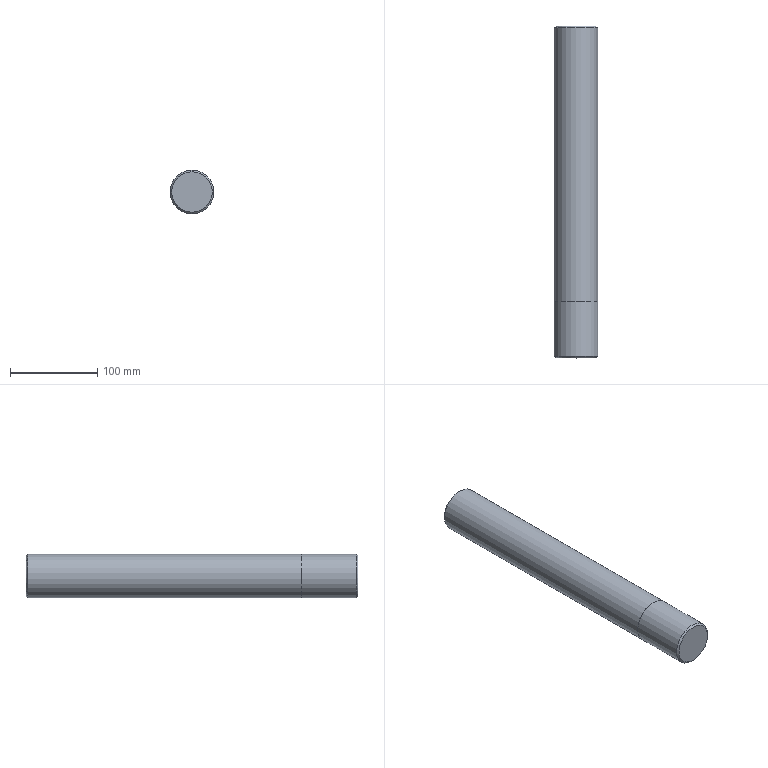Component | NX | GUIDE_PILLER | 1 solid | 7 faces | box 50.2 x 380 x 50.2 mm | volume 746538 mm3 | plane 3 | cylinder 2 | cone 2 | commonest cylinder face diameters 50.2 x1 50 x1
STEP:
#1=CARTESIAN_POINT('',(0.,0.,0.));
#2=DIRECTION('',(0.,0.,1.));
#3=DIRECTION('',(1.,0.,0.));
#4=AXIS2_PLACEMENT_3D('',#1,#2,#3);
#5=CARTESIAN_POINT('',(-120.,-68.,-232.946));
#6=VERTEX_POINT('',#5);
#7=CARTESIAN_POINT('',(-120.,-68.,-182.746));
#8=VERTEX_POINT('',#7);
#9=CARTESIAN_POINT('',(-120.,-68.,-207.846));
#10=DIRECTION('',(0.,1.,0.));
#11=DIRECTION('',(0.,0.,-1.));
#12=AXIS2_PLACEMENT_3D('',#9,#10,#11);
#13=CIRCLE('',#12,25.1);
#14=CARTESIAN_POINT('',(-120.,310.,-207.846));
#15=DIRECTION('',(0.,-1.,-0.));
#16=DIRECTION('',(0.,-0.,1.));
#17=AXIS2_PLACEMENT_3D('',#14,#15,#16);
#18=CYLINDRICAL_SURFACE('',#17,25.1);
#19=CARTESIAN_POINT('',(3.142,378.));
#20=DIRECTION('',(-1.,0.));
#21=VECTOR('',#20,1.);
#22=LINE('',#19,#21);
#23=(GEOMETRIC_REPRESENTATION_CONTEXT(2)PARAMETRIC_REPRESENTATION_CONTEXT()REPRESENTATION_CONTEXT('',''));
#24=DEFINITIONAL_REPRESENTATION('',(#22),#23);
#25=PCURVE('',#18,#24);
#26=CARTESIAN_POINT('',(-120.,-70.,-207.846));
#27=DIRECTION('',(0.,1.,0.));
#28=DIRECTION('',(0.,0.,-1.));
#29=AXIS2_PLACEMENT_3D('',#26,#27,#28);
#30=CONICAL_SURFACE('',#29,23.1,0.7854);
#31=CARTESIAN_POINT('',(0.,2.));
#32=DIRECTION('',(1.,0.));
#33=VECTOR('',#32,1.);
#34=LINE('',#31,#33);
#35=(GEOMETRIC_REPRESENTATION_CONTEXT(2)PARAMETRIC_REPRESENTATION_CONTEXT()REPRESENTATION_CONTEXT('',''));
#36=DEFINITIONAL_REPRESENTATION('',(#34),#35);
#37=PCURVE('',#30,#36);
#38=SURFACE_CURVE('',#13,(#25,#37),.PCURVE_S1.);
#39=EDGE_CURVE('',#6,#8,#38,.T.);
#40=ORIENTED_EDGE('',*,*,#39,.T.);
#41=CARTESIAN_POINT('',(-120.,-5.,-182.746));
#42=VERTEX_POINT('',#41);
#43=CARTESIAN_POINT('',(-120.,-5.,-182.746));
#44=CARTESIAN_POINT('',(-120.,-68.,-182.746));
#45=B_SPLINE_CURVE_WITH_KNOTS('',1,(#43,#44),.UNSPECIFIED.,.F.,.F.,(2,2),(315.,378.),.PIECEWISE_BEZIER_KNOTS.);
#46=CARTESIAN_POINT('',(0.,0.));
#47=DIRECTION('',(0.,1.));
#48=VECTOR('',#47,1.);
#49=LINE('',#46,#48);
#50=(GEOMETRIC_REPRESENTATION_CONTEXT(2)PARAMETRIC_REPRESENTATION_CONTEXT()REPRESENTATION_CONTEXT('',''));
#51=DEFINITIONAL_REPRESENTATION('',(#49),#50);
#52=PCURVE('',#18,#51);
#53=CARTESIAN_POINT('',(6.283,0.));
#54=DIRECTION('',(0.,1.));
#55=VECTOR('',#54,1.);
#56=LINE('',#53,#55);
#57=(GEOMETRIC_REPRESENTATION_CONTEXT(2)PARAMETRIC_REPRESENTATION_CONTEXT()REPRESENTATION_CONTEXT('',''));
#58=DEFINITIONAL_REPRESENTATION('',(#56),#57);
#59=PCURVE('',#18,#58);
#60=SEAM_CURVE('',#45,(#52,#59),.PCURVE_S1.);
#61=EDGE_CURVE('',#42,#8,#60,.T.);
#62=ORIENTED_EDGE('',*,*,#61,.F.);
#63=CARTESIAN_POINT('',(-120.,-5.,-207.846));
#64=DIRECTION('',(0.,-1.,-0.));
#65=DIRECTION('',(0.,-0.,1.));
#66=AXIS2_PLACEMENT_3D('',#63,#64,#65);
#67=CIRCLE('',#66,25.1);
#68=CARTESIAN_POINT('',(0.,315.));
#69=DIRECTION('',(1.,0.));
#70=VECTOR('',#69,1.);
#71=LINE('',#68,#70);
#72=(GEOMETRIC_REPRESENTATION_CONTEXT(2)PARAMETRIC_REPRESENTATION_CONTEXT()REPRESENTATION_CONTEXT('',''));
#73=DEFINITIONAL_REPRESENTATION('',(#71),#72);
#74=PCURVE('',#18,#73);
#75=CARTESIAN_POINT('',(-120.,-5.,-182.846));
#76=DIRECTION('',(0.,-1.,-0.));
#77=DIRECTION('',(0.,-0.,1.));
#78=AXIS2_PLACEMENT_3D('',#75,#76,#77);
#79=PLANE('',#78);
#80=CARTESIAN_POINT('',(-25.,0.));
#81=DIRECTION('',(1.,0.));
#82=AXIS2_PLACEMENT_2D('',#80,#81);
#83=CIRCLE('',#82,25.1);
#84=(GEOMETRIC_REPRESENTATION_CONTEXT(2)PARAMETRIC_REPRESENTATION_CONTEXT()REPRESENTATION_CONTEXT('',''));
#85=DEFINITIONAL_REPRESENTATION('',(#83),#84);
#86=PCURVE('',#79,#85);
#87=SURFACE_CURVE('',#67,(#74,#86),.PCURVE_S1.);
#88=EDGE_CURVE('',#42,#42,#87,.T.);
#89=ORIENTED_EDGE('',*,*,#88,.T.);
#90=ORIENTED_EDGE('',*,*,#61,.T.);
#91=CARTESIAN_POINT('',(-120.,-68.,-207.846));
#92=DIRECTION('',(0.,1.,0.));
#93=DIRECTION('',(0.,0.,-1.));
#94=AXIS2_PLACEMENT_3D('',#91,#92,#93);
#95=CIRCLE('',#94,25.1);
#96=CARTESIAN_POINT('',(9.425,378.));
#97=DIRECTION('',(-1.,0.));
#98=VECTOR('',#97,1.);
#99=LINE('',#96,#98);
#100=(GEOMETRIC_REPRESENTATION_CONTEXT(2)PARAMETRIC_REPRESENTATION_CONTEXT()REPRESENTATION_CONTEXT('',''));
#101=DEFINITIONAL_REPRESENTATION('',(#99),#100);
#102=PCURVE('',#18,#101);
#103=CARTESIAN_POINT('',(0.,2.));
#104=DIRECTION('',(1.,0.));
#105=VECTOR('',#104,1.);
#106=LINE('',#103,#105);
#107=(GEOMETRIC_REPRESENTATION_CONTEXT(2)PARAMETRIC_REPRESENTATION_CONTEXT()REPRESENTATION_CONTEXT('',''));
#108=DEFINITIONAL_REPRESENTATION('',(#106),#107);
#109=PCURVE('',#30,#108);
#110=SURFACE_CURVE('',#95,(#102,#109),.PCURVE_S1.);
#111=EDGE_CURVE('',#8,#6,#110,.T.);
#112=ORIENTED_EDGE('',*,*,#111,.T.);
#113=EDGE_LOOP('',(#40,#62,#89,#90,#112));
#114=FACE_BOUND('',#113,.T.);
#115=ADVANCED_FACE('',(#114),#18,.T.);
#116=CARTESIAN_POINT('',(-120.,-70.,-230.946));
#117=VERTEX_POINT('',#116);
#118=CARTESIAN_POINT('',(-120.,-70.,-207.846));
#119=DIRECTION('',(0.,-1.,-0.));
#120=DIRECTION('',(0.,0.,-1.));
#121=AXIS2_PLACEMENT_3D('',#118,#119,#120);
#122=CIRCLE('',#121,23.1);
#123=CARTESIAN_POINT('',(-120.,-70.,-182.746));
#124=DIRECTION('',(0.,1.,0.));
#125=DIRECTION('',(0.,0.,-1.));
#126=AXIS2_PLACEMENT_3D('',#123,#124,#125);
#127=PLANE('',#126);
#128=CARTESIAN_POINT('',(48.2,0.));
#129=CARTESIAN_POINT('',(48.2,-40.01));
#130=CARTESIAN_POINT('',(13.55,-20.005));
#131=CARTESIAN_POINT('',(-21.1,-0.));
#132=CARTESIAN_POINT('',(13.55,20.005));
#133=CARTESIAN_POINT('',(48.2,40.01));
#134=CARTESIAN_POINT('',(48.2,0.));
#135=(BOUNDED_CURVE()B_SPLINE_CURVE(2,(#128,#129,#130,#131,#132,#133,#134),.UNSPECIFIED.,.T.,.F.)B_SPLINE_CURVE_WITH_KNOTS((1,2,2,2,2,1),(-2.094,0.,2.094,4.189,6.283,8.378),.UNSPECIFIED.)CURVE()GEOMETRIC_REPRESENTATION_ITEM()RATIONAL_B_SPLINE_CURVE((1.,0.5,1.,0.5,1.,0.5,1.))REPRESENTATION_ITEM(''));
#136=(GEOMETRIC_REPRESENTATION_CONTEXT(2)PARAMETRIC_REPRESENTATION_CONTEXT()REPRESENTATION_CONTEXT('',''));
#137=DEFINITIONAL_REPRESENTATION('',(#135),#136);
#138=PCURVE('',#127,#137);
#139=CARTESIAN_POINT('',(6.283,-0.));
#140=DIRECTION('',(-1.,0.));
#141=VECTOR('',#140,1.);
#142=LINE('',#139,#141);
#143=(GEOMETRIC_REPRESENTATION_CONTEXT(2)PARAMETRIC_REPRESENTATION_CONTEXT()REPRESENTATION_CONTEXT('',''));
#144=DEFINITIONAL_REPRESENTATION('',(#142),#143);
#145=PCURVE('',#30,#144);
#146=SURFACE_CURVE('',#122,(#138,#145),.PCURVE_S1.);
#147=EDGE_CURVE('',#117,#117,#146,.T.);
#148=ORIENTED_EDGE('',*,*,#147,.T.);
#149=EDGE_LOOP('',(#148));
#150=FACE_BOUND('',#149,.T.);
#151=ADVANCED_FACE('',(#150),#127,.F.);
#152=CARTESIAN_POINT('',(-120.,310.,-184.846));
#153=VERTEX_POINT('',#152);
#154=CARTESIAN_POINT('',(-120.,310.,-207.846));
#155=DIRECTION('',(0.,1.,0.));
#156=DIRECTION('',(0.,-0.,1.));
#157=AXIS2_PLACEMENT_3D('',#154,#155,#156);
#158=CIRCLE('',#157,23.);
#159=CARTESIAN_POINT('',(-120.,310.,-207.846));
#160=DIRECTION('',(0.,-1.,-0.));
#161=DIRECTION('',(0.,-0.,1.));
#162=AXIS2_PLACEMENT_3D('',#159,#160,#161);
#163=PLANE('',#162);
#164=CARTESIAN_POINT('',(23.,0.));
#165=CARTESIAN_POINT('',(23.,-39.837));
#166=CARTESIAN_POINT('',(-11.5,-19.919));
#167=CARTESIAN_POINT('',(-46.,-0.));
#168=CARTESIAN_POINT('',(-11.5,19.919));
#169=CARTESIAN_POINT('',(23.,39.837));
#170=CARTESIAN_POINT('',(23.,0.));
#171=(BOUNDED_CURVE()B_SPLINE_CURVE(2,(#164,#165,#166,#167,#168,#169,#170),.UNSPECIFIED.,.T.,.F.)B_SPLINE_CURVE_WITH_KNOTS((1,2,2,2,2,1),(-2.094,0.,2.094,4.189,6.283,8.378),.UNSPECIFIED.)CURVE()GEOMETRIC_REPRESENTATION_ITEM()RATIONAL_B_SPLINE_CURVE((1.,0.5,1.,0.5,1.,0.5,1.))REPRESENTATION_ITEM(''));
#172=(GEOMETRIC_REPRESENTATION_CONTEXT(2)PARAMETRIC_REPRESENTATION_CONTEXT()REPRESENTATION_CONTEXT('',''));
#173=DEFINITIONAL_REPRESENTATION('',(#171),#172);
#174=PCURVE('',#163,#173);
#175=CARTESIAN_POINT('',(-120.,308.,-207.846));
#176=DIRECTION('',(0.,-1.,-0.));
#177=DIRECTION('',(0.,-0.,1.));
#178=AXIS2_PLACEMENT_3D('',#175,#176,#177);
#179=CONICAL_SURFACE('',#178,25.,0.7854);
#180=CARTESIAN_POINT('',(6.283,-2.));
#181=DIRECTION('',(-1.,0.));
#182=VECTOR('',#181,1.);
#183=LINE('',#180,#182);
#184=(GEOMETRIC_REPRESENTATION_CONTEXT(2)PARAMETRIC_REPRESENTATION_CONTEXT()REPRESENTATION_CONTEXT('',''));
#185=DEFINITIONAL_REPRESENTATION('',(#183),#184);
#186=PCURVE('',#179,#185);
#187=SURFACE_CURVE('',#158,(#174,#186),.PCURVE_S1.);
#188=EDGE_CURVE('',#153,#153,#187,.T.);
#189=ORIENTED_EDGE('',*,*,#188,.T.);
#190=EDGE_LOOP('',(#189));
#191=FACE_BOUND('',#190,.T.);
#192=ADVANCED_FACE('',(#191),#163,.F.);
#193=CARTESIAN_POINT('',(-120.,308.,-182.846));
#194=VERTEX_POINT('',#193);
#195=CARTESIAN_POINT('',(-120.,308.,-207.846));
#196=DIRECTION('',(0.,-1.,-0.));
#197=DIRECTION('',(0.,-0.,1.));
#198=AXIS2_PLACEMENT_3D('',#195,#196,#197);
#199=CIRCLE('',#198,25.);
#200=CARTESIAN_POINT('',(-120.,310.,-207.846));
#201=DIRECTION('',(0.,-1.,-0.));
#202=DIRECTION('',(0.,-0.,1.));
#203=AXIS2_PLACEMENT_3D('',#200,#201,#202);
#204=CYLINDRICAL_SURFACE('',#203,25.);
#205=CARTESIAN_POINT('',(0.,2.));
#206=DIRECTION('',(1.,0.));
#207=VECTOR('',#206,1.);
#208=LINE('',#205,#207);
#209=(GEOMETRIC_REPRESENTATION_CONTEXT(2)PARAMETRIC_REPRESENTATION_CONTEXT()REPRESENTATION_CONTEXT('',''));
#210=DEFINITIONAL_REPRESENTATION('',(#208),#209);
#211=PCURVE('',#204,#210);
#212=CARTESIAN_POINT('',(0.,0.));
#213=DIRECTION('',(1.,0.));
#214=VECTOR('',#213,1.);
#215=LINE('',#212,#214);
#216=(GEOMETRIC_REPRESENTATION_CONTEXT(2)PARAMETRIC_REPRESENTATION_CONTEXT()REPRESENTATION_CONTEXT('',''));
#217=DEFINITIONAL_REPRESENTATION('',(#215),#216);
#218=PCURVE('',#179,#217);
#219=SURFACE_CURVE('',#199,(#211,#218),.PCURVE_S1.);
#220=EDGE_CURVE('',#194,#194,#219,.T.);
#221=ORIENTED_EDGE('',*,*,#220,.T.);
#222=CARTESIAN_POINT('',(-120.,-5.,-182.846));
#223=VERTEX_POINT('',#222);
#224=CARTESIAN_POINT('',(-120.,308.,-182.846));
#225=CARTESIAN_POINT('',(-120.,-5.,-182.846));
#226=B_SPLINE_CURVE_WITH_KNOTS('',1,(#224,#225),.UNSPECIFIED.,.F.,.F.,(2,2),(2.,315.),.PIECEWISE_BEZIER_KNOTS.);
#227=CARTESIAN_POINT('',(6.283,0.));
#228=DIRECTION('',(0.,1.));
#229=VECTOR('',#228,1.);
#230=LINE('',#227,#229);
#231=(GEOMETRIC_REPRESENTATION_CONTEXT(2)PARAMETRIC_REPRESENTATION_CONTEXT()REPRESENTATION_CONTEXT('',''));
#232=DEFINITIONAL_REPRESENTATION('',(#230),#231);
#233=PCURVE('',#204,#232);
#234=CARTESIAN_POINT('',(0.,0.));
#235=DIRECTION('',(0.,1.));
#236=VECTOR('',#235,1.);
#237=LINE('',#234,#236);
#238=(GEOMETRIC_REPRESENTATION_CONTEXT(2)PARAMETRIC_REPRESENTATION_CONTEXT()REPRESENTATION_CONTEXT('',''));
#239=DEFINITIONAL_REPRESENTATION('',(#237),#238);
#240=PCURVE('',#204,#239);
#241=SEAM_CURVE('',#226,(#233,#240),.PCURVE_S1.);
#242=EDGE_CURVE('',#194,#223,#241,.T.);
#243=ORIENTED_EDGE('',*,*,#242,.T.);
#244=CARTESIAN_POINT('',(-120.,-5.,-207.846));
#245=DIRECTION('',(0.,-1.,-0.));
#246=DIRECTION('',(0.,-0.,1.));
#247=AXIS2_PLACEMENT_3D('',#244,#245,#246);
#248=CIRCLE('',#247,25.);
#249=CARTESIAN_POINT('',(0.,315.));
#250=DIRECTION('',(1.,0.));
#251=VECTOR('',#250,1.);
#252=LINE('',#249,#251);
#253=(GEOMETRIC_REPRESENTATION_CONTEXT(2)PARAMETRIC_REPRESENTATION_CONTEXT()REPRESENTATION_CONTEXT('',''));
#254=DEFINITIONAL_REPRESENTATION('',(#252),#253);
#255=PCURVE('',#204,#254);
#256=CARTESIAN_POINT('',(-25.,0.));
#257=DIRECTION('',(1.,0.));
#258=AXIS2_PLACEMENT_2D('',#256,#257);
#259=CIRCLE('',#258,25.);
#260=(GEOMETRIC_REPRESENTATION_CONTEXT(2)PARAMETRIC_REPRESENTATION_CONTEXT()REPRESENTATION_CONTEXT('',''));
#261=DEFINITIONAL_REPRESENTATION('',(#259),#260);
#262=PCURVE('',#79,#261);
#263=SURFACE_CURVE('',#248,(#255,#262),.PCURVE_S1.);
#264=EDGE_CURVE('',#223,#223,#263,.T.);
#265=ORIENTED_EDGE('',*,*,#264,.F.);
#266=ORIENTED_EDGE('',*,*,#242,.F.);
#267=EDGE_LOOP('',(#221,#243,#265,#266));
#268=FACE_BOUND('',#267,.T.);
#269=ADVANCED_FACE('',(#268),#204,.T.);
#270=ORIENTED_EDGE('',*,*,#88,.F.);
#271=EDGE_LOOP('',(#270));
#272=FACE_BOUND('',#271,.T.);
#273=ORIENTED_EDGE('',*,*,#264,.T.);
#274=EDGE_LOOP('',(#273));
#275=FACE_BOUND('',#274,.T.);
#276=ADVANCED_FACE('',(#272,#275),#79,.F.);
#277=ORIENTED_EDGE('',*,*,#39,.F.);
#278=CARTESIAN_POINT('',(-120.,-70.,-230.946));
#279=CARTESIAN_POINT('',(-120.,-68.,-232.946));
#280=B_SPLINE_CURVE_WITH_KNOTS('',1,(#278,#279),.UNSPECIFIED.,.F.,.F.,(2,2),(-0.,2.828),.PIECEWISE_BEZIER_KNOTS.);
#281=CARTESIAN_POINT('',(0.,0.));
#282=DIRECTION('',(0.,1.));
#283=VECTOR('',#282,1.);
#284=LINE('',#281,#283);
#285=(GEOMETRIC_REPRESENTATION_CONTEXT(2)PARAMETRIC_REPRESENTATION_CONTEXT()REPRESENTATION_CONTEXT('',''));
#286=DEFINITIONAL_REPRESENTATION('',(#284),#285);
#287=PCURVE('',#30,#286);
#288=CARTESIAN_POINT('',(6.283,0.));
#289=DIRECTION('',(0.,1.));
#290=VECTOR('',#289,1.);
#291=LINE('',#288,#290);
#292=(GEOMETRIC_REPRESENTATION_CONTEXT(2)PARAMETRIC_REPRESENTATION_CONTEXT()REPRESENTATION_CONTEXT('',''));
#293=DEFINITIONAL_REPRESENTATION('',(#291),#292);
#294=PCURVE('',#30,#293);
#295=SEAM_CURVE('',#280,(#287,#294),.PCURVE_S1.);
#296=EDGE_CURVE('',#117,#6,#295,.T.);
#297=ORIENTED_EDGE('',*,*,#296,.F.);
#298=ORIENTED_EDGE('',*,*,#147,.F.);
#299=ORIENTED_EDGE('',*,*,#296,.T.);
#300=ORIENTED_EDGE('',*,*,#111,.F.);
#301=EDGE_LOOP('',(#277,#297,#298,#299,#300));
#302=FACE_BOUND('',#301,.T.);
#303=ADVANCED_FACE('',(#302),#30,.T.);
#304=ORIENTED_EDGE('',*,*,#188,.F.);
#305=CARTESIAN_POINT('',(-120.,310.,-184.846));
#306=CARTESIAN_POINT('',(-120.,308.,-182.846));
#307=B_SPLINE_CURVE_WITH_KNOTS('',1,(#305,#306),.UNSPECIFIED.,.F.,.F.,(2,2),(-2.828,0.),.PIECEWISE_BEZIER_KNOTS.);
#308=CARTESIAN_POINT('',(6.283,0.));
#309=DIRECTION('',(0.,1.));
#310=VECTOR('',#309,1.);
#311=LINE('',#308,#310);
#312=(GEOMETRIC_REPRESENTATION_CONTEXT(2)PARAMETRIC_REPRESENTATION_CONTEXT()REPRESENTATION_CONTEXT('',''));
#313=DEFINITIONAL_REPRESENTATION('',(#311),#312);
#314=PCURVE('',#179,#313);
#315=CARTESIAN_POINT('',(0.,0.));
#316=DIRECTION('',(0.,1.));
#317=VECTOR('',#316,1.);
#318=LINE('',#315,#317);
#319=(GEOMETRIC_REPRESENTATION_CONTEXT(2)PARAMETRIC_REPRESENTATION_CONTEXT()REPRESENTATION_CONTEXT('',''));
#320=DEFINITIONAL_REPRESENTATION('',(#318),#319);
#321=PCURVE('',#179,#320);
#322=SEAM_CURVE('',#307,(#314,#321),.PCURVE_S1.);
#323=EDGE_CURVE('',#153,#194,#322,.T.);
#324=ORIENTED_EDGE('',*,*,#323,.T.);
#325=ORIENTED_EDGE('',*,*,#220,.F.);
#326=ORIENTED_EDGE('',*,*,#323,.F.);
#327=EDGE_LOOP('',(#304,#324,#325,#326));
#328=FACE_BOUND('',#327,.T.);
#329=ADVANCED_FACE('',(#328),#179,.T.);
#330=CLOSED_SHELL('',(#115,#151,#192,#269,#276,#303,#329));
#331=MANIFOLD_SOLID_BREP('',#330);
#332=(LENGTH_UNIT()NAMED_UNIT(*)SI_UNIT(.MILLI.,.METRE.));
#333=UNCERTAINTY_MEASURE_WITH_UNIT(LENGTH_MEASURE(0.00001),#332,'','');
#334=(NAMED_UNIT(*)PLANE_ANGLE_UNIT()SI_UNIT($,.RADIAN.));
#335=(NAMED_UNIT(*)SI_UNIT($,.STERADIAN.)SOLID_ANGLE_UNIT());
#336=(GEOMETRIC_REPRESENTATION_CONTEXT(3)GLOBAL_UNCERTAINTY_ASSIGNED_CONTEXT((#333))GLOBAL_UNIT_ASSIGNED_CONTEXT((#332,#334,#335))REPRESENTATION_CONTEXT('',''));
#337=ADVANCED_BREP_SHAPE_REPRESENTATION('',(#4,#331),#336);